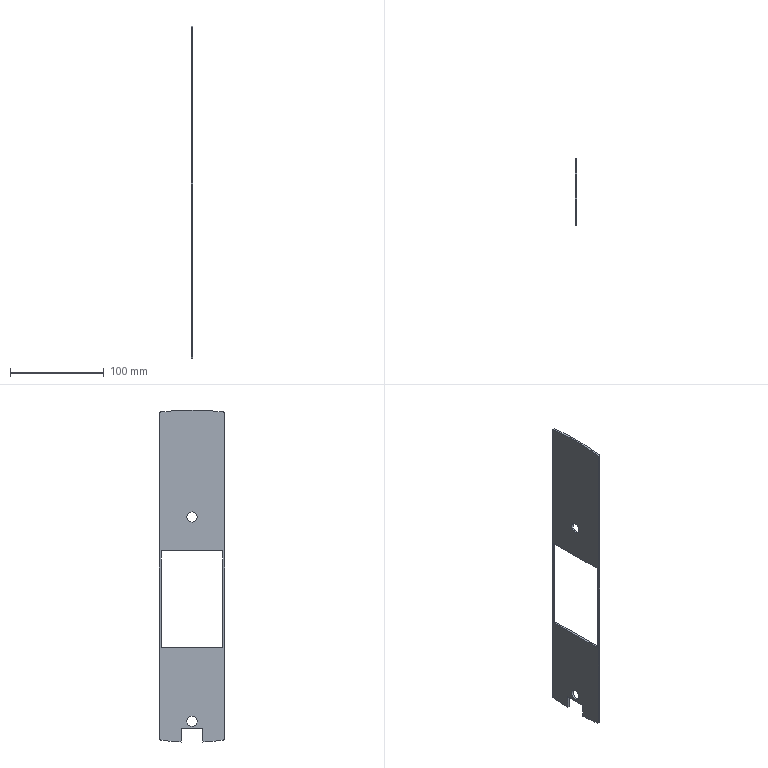Component | NX | FIXING_PLATE | 1 solid | 20 faces | volume 34815 mm3 | plane 11 | cylinder 9 | commonest cylinder face diameters 4 x4 466.75 x3 10.945 x2